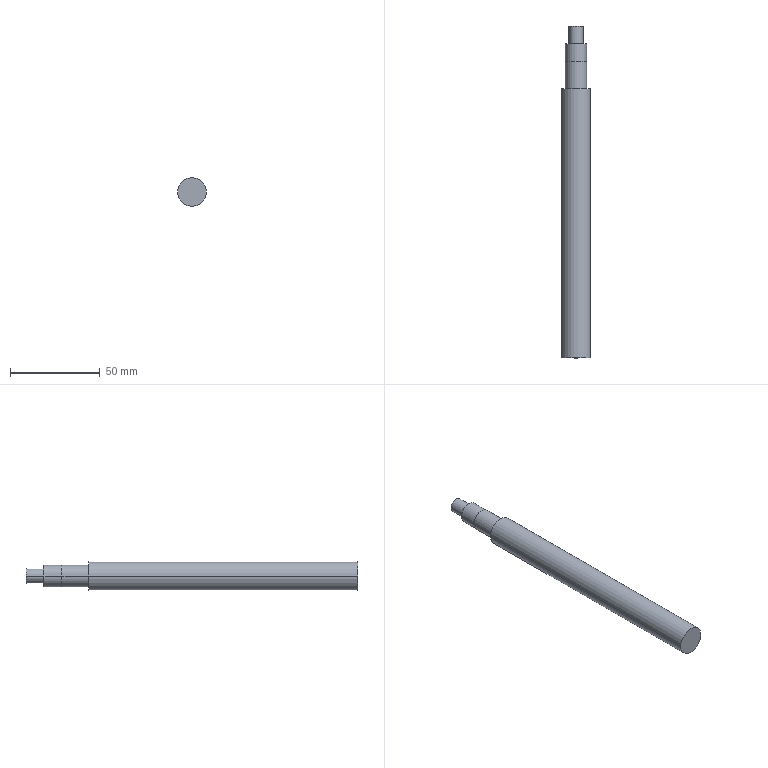Component | SolidWorks | FeedingPressingScrew1-1-1 | 1 solid | 13 faces | box 16 x 185 x 16 mm | volume 33452 mm3 | cylinder 8 | plane 5 | commonest cylinder face diameters 8 x2 11.8 x2 12 x2 16 x2
build123d program:
from build123d import *

# Parameters (mm, degrees)
SKETCH1_R           = 8
BOSS_EXTRUDE1_DEPTH = 150
SKETCH2_R           = 6
BOSS_EXTRUDE2_DEPTH = 15
SKETCH3_R           = 5.9
BOSS_EXTRUDE3_DEPTH = 10
SKETCH4_R           = 4
BOSS_EXTRUDE4_DEPTH = 10


with BuildPart() as part:
    # Sketch1 → Boss-Extrude1 (new body)
    with BuildSketch(Plane.XY):
        Circle(SKETCH1_R)
    extrude(amount=BOSS_EXTRUDE1_DEPTH)

    # Sketch2 → Boss-Extrude2 (add)
    with BuildSketch(Plane.XY.offset(150)):
        with Locations(Location((0, 0, 0), (0, 0, 180))):
            Circle(SKETCH2_R)
    extrude(amount=BOSS_EXTRUDE2_DEPTH)

    # Sketch3 → Boss-Extrude3 (add)
    with BuildSketch(Plane.XY.offset(165)):
        Circle(SKETCH3_R)
    extrude(amount=BOSS_EXTRUDE3_DEPTH)

    # Sketch4 → Boss-Extrude4 (add)
    with BuildSketch(Plane.XY.offset(175)):
        Circle(SKETCH4_R)
    extrude(amount=BOSS_EXTRUDE4_DEPTH)


solid = part.part

# Placed as in the assembly
solid = solid.moved(Location((4.873, 348, 588.209), (-90, 0, 0)))
STEP:
#1=COLOUR_RGB('',0.7922,0.8196,0.9333);
#2=FILL_AREA_STYLE_COLOUR('',#1);
#3=FILL_AREA_STYLE('',(#2));
#4=SURFACE_STYLE_FILL_AREA(#3);
#5=SURFACE_SIDE_STYLE('',(#4));
#6=SURFACE_STYLE_USAGE(.BOTH.,#5);
#7=PRESENTATION_STYLE_ASSIGNMENT((#6));
#8=CARTESIAN_POINT('',(0.3493,20.984,23.158));
#9=VERTEX_POINT('',#8);
#10=CARTESIAN_POINT('',(0.03438,20.984,23.158));
#11=VERTEX_POINT('',#10);
#12=CARTESIAN_POINT('',(0.1919,20.984,23.158));
#13=DIRECTION('',(0.,1.,0.));
#14=DIRECTION('',(1.,0.,0.));
#15=AXIS2_PLACEMENT_3D('',#12,#13,#14);
#16=CIRCLE('',#15,0.1575);
#17=EDGE_CURVE('',#9,#11,#16,.T.);
#18=ORIENTED_EDGE('',*,*,#17,.F.);
#19=CARTESIAN_POINT('',(0.3493,20.591,23.158));
#20=VERTEX_POINT('',#19);
#21=CARTESIAN_POINT('',(0.3493,20.984,23.158));
#22=DIRECTION('',(-0.,-1.,-0.));
#23=VECTOR('',#22,39.37);
#24=LINE('',#21,#23);
#25=EDGE_CURVE('',#9,#20,#24,.T.);
#26=ORIENTED_EDGE('',*,*,#25,.T.);
#27=CARTESIAN_POINT('',(0.03438,20.591,23.158));
#28=VERTEX_POINT('',#27);
#29=CARTESIAN_POINT('',(0.1919,20.591,23.158));
#30=DIRECTION('',(0.,1.,0.));
#31=DIRECTION('',(1.,0.,0.));
#32=AXIS2_PLACEMENT_3D('',#29,#30,#31);
#33=CIRCLE('',#32,0.1575);
#34=EDGE_CURVE('',#20,#28,#33,.T.);
#35=ORIENTED_EDGE('',*,*,#34,.T.);
#36=CARTESIAN_POINT('',(0.03438,20.984,23.158));
#37=DIRECTION('',(-0.,-1.,-0.));
#38=VECTOR('',#37,39.37);
#39=LINE('',#36,#38);
#40=EDGE_CURVE('',#11,#28,#39,.T.);
#41=ORIENTED_EDGE('',*,*,#40,.F.);
#42=EDGE_LOOP('',(#18,#26,#35,#41));
#43=FACE_OUTER_BOUND('',#42,.T.);
#44=CARTESIAN_POINT('',(0.1919,20.984,23.158));
#45=DIRECTION('',(-0.,-1.,-0.));
#46=DIRECTION('',(-1.,0.,0.));
#47=AXIS2_PLACEMENT_3D('',#44,#45,#46);
#48=CYLINDRICAL_SURFACE('',#47,0.1575);
#49=ADVANCED_FACE('',(#43),#48,.T.);
#50=CARTESIAN_POINT('',(0.4241,20.591,23.158));
#51=VERTEX_POINT('',#50);
#52=CARTESIAN_POINT('',(-0.04043,20.591,23.158));
#53=VERTEX_POINT('',#52);
#54=CARTESIAN_POINT('',(0.1919,20.591,23.158));
#55=DIRECTION('',(0.,1.,0.));
#56=DIRECTION('',(1.,0.,0.));
#57=AXIS2_PLACEMENT_3D('',#54,#55,#56);
#58=CIRCLE('',#57,0.2323);
#59=EDGE_CURVE('',#51,#53,#58,.T.);
#60=ORIENTED_EDGE('',*,*,#59,.F.);
#61=CARTESIAN_POINT('',(0.4241,20.197,23.158));
#62=VERTEX_POINT('',#61);
#63=CARTESIAN_POINT('',(0.4241,20.591,23.158));
#64=DIRECTION('',(-0.,-1.,-0.));
#65=VECTOR('',#64,39.37);
#66=LINE('',#63,#65);
#67=EDGE_CURVE('',#51,#62,#66,.T.);
#68=ORIENTED_EDGE('',*,*,#67,.T.);
#69=CARTESIAN_POINT('',(-0.04043,20.197,23.158));
#70=VERTEX_POINT('',#69);
#71=CARTESIAN_POINT('',(0.1919,20.197,23.158));
#72=DIRECTION('',(0.,1.,0.));
#73=DIRECTION('',(1.,0.,0.));
#74=AXIS2_PLACEMENT_3D('',#71,#72,#73);
#75=CIRCLE('',#74,0.2323);
#76=EDGE_CURVE('',#62,#70,#75,.T.);
#77=ORIENTED_EDGE('',*,*,#76,.T.);
#78=CARTESIAN_POINT('',(-0.04043,20.591,23.158));
#79=DIRECTION('',(-0.,-1.,-0.));
#80=VECTOR('',#79,39.37);
#81=LINE('',#78,#80);
#82=EDGE_CURVE('',#53,#70,#81,.T.);
#83=ORIENTED_EDGE('',*,*,#82,.F.);
#84=EDGE_LOOP('',(#60,#68,#77,#83));
#85=FACE_OUTER_BOUND('',#84,.T.);
#86=CARTESIAN_POINT('',(0.1919,20.591,23.158));
#87=DIRECTION('',(-0.,-1.,-0.));
#88=DIRECTION('',(-1.,0.,0.));
#89=AXIS2_PLACEMENT_3D('',#86,#87,#88);
#90=CYLINDRICAL_SURFACE('',#89,0.2323);
#91=ADVANCED_FACE('',(#85),#90,.T.);
#92=CARTESIAN_POINT('',(0.4281,20.197,23.158));
#93=VERTEX_POINT('',#92);
#94=CARTESIAN_POINT('',(-0.04436,20.197,23.158));
#95=VERTEX_POINT('',#94);
#96=CARTESIAN_POINT('',(0.1919,20.197,23.158));
#97=DIRECTION('',(0.,1.,0.));
#98=DIRECTION('',(1.,0.,0.));
#99=AXIS2_PLACEMENT_3D('',#96,#97,#98);
#100=CIRCLE('',#99,0.2362);
#101=EDGE_CURVE('',#93,#95,#100,.T.);
#102=ORIENTED_EDGE('',*,*,#101,.F.);
#103=CARTESIAN_POINT('',(0.4281,19.606,23.158));
#104=VERTEX_POINT('',#103);
#105=CARTESIAN_POINT('',(0.4281,20.197,23.158));
#106=DIRECTION('',(-0.,-1.,-0.));
#107=VECTOR('',#106,39.37);
#108=LINE('',#105,#107);
#109=EDGE_CURVE('',#93,#104,#108,.T.);
#110=ORIENTED_EDGE('',*,*,#109,.T.);
#111=CARTESIAN_POINT('',(-0.04436,19.606,23.158));
#112=VERTEX_POINT('',#111);
#113=CARTESIAN_POINT('',(0.1919,19.606,23.158));
#114=DIRECTION('',(0.,1.,0.));
#115=DIRECTION('',(1.,0.,0.));
#116=AXIS2_PLACEMENT_3D('',#113,#114,#115);
#117=CIRCLE('',#116,0.2362);
#118=EDGE_CURVE('',#104,#112,#117,.T.);
#119=ORIENTED_EDGE('',*,*,#118,.T.);
#120=CARTESIAN_POINT('',(-0.04436,20.197,23.158));
#121=DIRECTION('',(-0.,-1.,-0.));
#122=VECTOR('',#121,39.37);
#123=LINE('',#120,#122);
#124=EDGE_CURVE('',#95,#112,#123,.T.);
#125=ORIENTED_EDGE('',*,*,#124,.F.);
#126=EDGE_LOOP('',(#102,#110,#119,#125));
#127=FACE_OUTER_BOUND('',#126,.T.);
#128=CARTESIAN_POINT('',(0.1919,20.197,23.158));
#129=DIRECTION('',(-0.,-1.,-0.));
#130=DIRECTION('',(-1.,0.,0.));
#131=AXIS2_PLACEMENT_3D('',#128,#129,#130);
#132=CYLINDRICAL_SURFACE('',#131,0.2362);
#133=ADVANCED_FACE('',(#127),#132,.T.);
#134=CARTESIAN_POINT('',(0.5068,19.606,23.158));
#135=VERTEX_POINT('',#134);
#136=CARTESIAN_POINT('',(-0.1231,19.606,23.158));
#137=VERTEX_POINT('',#136);
#138=CARTESIAN_POINT('',(0.1919,19.606,23.158));
#139=DIRECTION('',(0.,1.,0.));
#140=DIRECTION('',(1.,0.,0.));
#141=AXIS2_PLACEMENT_3D('',#138,#139,#140);
#142=CIRCLE('',#141,0.315);
#143=EDGE_CURVE('',#135,#137,#142,.T.);
#144=ORIENTED_EDGE('',*,*,#143,.F.);
#145=CARTESIAN_POINT('',(0.5068,13.701,23.158));
#146=VERTEX_POINT('',#145);
#147=CARTESIAN_POINT('',(0.5068,19.606,23.158));
#148=DIRECTION('',(-0.,-1.,-0.));
#149=VECTOR('',#148,39.37);
#150=LINE('',#147,#149);
#151=EDGE_CURVE('',#135,#146,#150,.T.);
#152=ORIENTED_EDGE('',*,*,#151,.T.);
#153=CARTESIAN_POINT('',(-0.1231,13.701,23.158));
#154=VERTEX_POINT('',#153);
#155=CARTESIAN_POINT('',(0.1919,13.701,23.158));
#156=DIRECTION('',(0.,1.,0.));
#157=DIRECTION('',(1.,0.,0.));
#158=AXIS2_PLACEMENT_3D('',#155,#156,#157);
#159=CIRCLE('',#158,0.315);
#160=EDGE_CURVE('',#146,#154,#159,.T.);
#161=ORIENTED_EDGE('',*,*,#160,.T.);
#162=CARTESIAN_POINT('',(-0.1231,19.606,23.158));
#163=DIRECTION('',(-0.,-1.,-0.));
#164=VECTOR('',#163,39.37);
#165=LINE('',#162,#164);
#166=EDGE_CURVE('',#137,#154,#165,.T.);
#167=ORIENTED_EDGE('',*,*,#166,.F.);
#168=EDGE_LOOP('',(#144,#152,#161,#167));
#169=FACE_OUTER_BOUND('',#168,.T.);
#170=CARTESIAN_POINT('',(0.1919,19.606,23.158));
#171=DIRECTION('',(-0.,-1.,-0.));
#172=DIRECTION('',(-1.,0.,0.));
#173=AXIS2_PLACEMENT_3D('',#170,#171,#172);
#174=CYLINDRICAL_SURFACE('',#173,0.315);
#175=ADVANCED_FACE('',(#169),#174,.T.);
#176=ORIENTED_EDGE('',*,*,#151,.F.);
#177=CARTESIAN_POINT('',(0.1919,19.606,23.158));
#178=DIRECTION('',(0.,1.,0.));
#179=DIRECTION('',(1.,0.,0.));
#180=AXIS2_PLACEMENT_3D('',#177,#178,#179);
#181=CIRCLE('',#180,0.315);
#182=EDGE_CURVE('',#137,#135,#181,.T.);
#183=ORIENTED_EDGE('',*,*,#182,.F.);
#184=ORIENTED_EDGE('',*,*,#166,.T.);
#185=CARTESIAN_POINT('',(0.1919,13.701,23.158));
#186=DIRECTION('',(0.,1.,0.));
#187=DIRECTION('',(1.,0.,0.));
#188=AXIS2_PLACEMENT_3D('',#185,#186,#187);
#189=CIRCLE('',#188,0.315);
#190=EDGE_CURVE('',#154,#146,#189,.T.);
#191=ORIENTED_EDGE('',*,*,#190,.T.);
#192=EDGE_LOOP('',(#176,#183,#184,#191));
#193=FACE_OUTER_BOUND('',#192,.T.);
#194=CARTESIAN_POINT('',(0.1919,19.606,23.158));
#195=DIRECTION('',(-0.,-1.,-0.));
#196=DIRECTION('',(-1.,0.,0.));
#197=AXIS2_PLACEMENT_3D('',#194,#195,#196);
#198=CYLINDRICAL_SURFACE('',#197,0.315);
#199=ADVANCED_FACE('',(#193),#198,.T.);
#200=CARTESIAN_POINT('',(0.1919,19.606,23.158));
#201=DIRECTION('',(0.,1.,0.));
#202=DIRECTION('',(1.,0.,0.));
#203=AXIS2_PLACEMENT_3D('',#200,#201,#202);
#204=CIRCLE('',#203,0.2362);
#205=EDGE_CURVE('',#112,#104,#204,.T.);
#206=ORIENTED_EDGE('',*,*,#205,.F.);
#207=ORIENTED_EDGE('',*,*,#118,.F.);
#208=EDGE_LOOP('',(#206,#207));
#209=FACE_BOUND('',#208,.T.);
#210=ORIENTED_EDGE('',*,*,#182,.T.);
#211=ORIENTED_EDGE('',*,*,#143,.T.);
#212=EDGE_LOOP('',(#210,#211));
#213=FACE_OUTER_BOUND('',#212,.T.);
#214=CARTESIAN_POINT('',(0.1919,19.606,23.158));
#215=DIRECTION('',(0.,1.,0.));
#216=DIRECTION('',(1.,-0.,-0.));
#217=AXIS2_PLACEMENT_3D('',#214,#215,#216);
#218=PLANE('',#217);
#219=ADVANCED_FACE('',(#209,#213),#218,.T.);
#220=ORIENTED_EDGE('',*,*,#190,.F.);
#221=ORIENTED_EDGE('',*,*,#160,.F.);
#222=EDGE_LOOP('',(#220,#221));
#223=FACE_OUTER_BOUND('',#222,.T.);
#224=CARTESIAN_POINT('',(0.1919,13.701,23.158));
#225=DIRECTION('',(0.,1.,0.));
#226=DIRECTION('',(1.,-0.,-0.));
#227=AXIS2_PLACEMENT_3D('',#224,#225,#226);
#228=PLANE('',#227);
#229=ADVANCED_FACE('',(#223),#228,.F.);
#230=ORIENTED_EDGE('',*,*,#109,.F.);
#231=CARTESIAN_POINT('',(0.1919,20.197,23.158));
#232=DIRECTION('',(0.,1.,0.));
#233=DIRECTION('',(1.,0.,0.));
#234=AXIS2_PLACEMENT_3D('',#231,#232,#233);
#235=CIRCLE('',#234,0.2362);
#236=EDGE_CURVE('',#95,#93,#235,.T.);
#237=ORIENTED_EDGE('',*,*,#236,.F.);
#238=ORIENTED_EDGE('',*,*,#124,.T.);
#239=ORIENTED_EDGE('',*,*,#205,.T.);
#240=EDGE_LOOP('',(#230,#237,#238,#239));
#241=FACE_OUTER_BOUND('',#240,.T.);
#242=CARTESIAN_POINT('',(0.1919,20.197,23.158));
#243=DIRECTION('',(-0.,-1.,-0.));
#244=DIRECTION('',(-1.,0.,0.));
#245=AXIS2_PLACEMENT_3D('',#242,#243,#244);
#246=CYLINDRICAL_SURFACE('',#245,0.2362);
#247=ADVANCED_FACE('',(#241),#246,.T.);
#248=CARTESIAN_POINT('',(0.1919,20.197,23.158));
#249=DIRECTION('',(0.,1.,0.));
#250=DIRECTION('',(1.,0.,0.));
#251=AXIS2_PLACEMENT_3D('',#248,#249,#250);
#252=CIRCLE('',#251,0.2323);
#253=EDGE_CURVE('',#70,#62,#252,.T.);
#254=ORIENTED_EDGE('',*,*,#253,.F.);
#255=ORIENTED_EDGE('',*,*,#76,.F.);
#256=EDGE_LOOP('',(#254,#255));
#257=FACE_BOUND('',#256,.T.);
#258=ORIENTED_EDGE('',*,*,#236,.T.);
#259=ORIENTED_EDGE('',*,*,#101,.T.);
#260=EDGE_LOOP('',(#258,#259));
#261=FACE_OUTER_BOUND('',#260,.T.);
#262=CARTESIAN_POINT('',(0.1919,20.197,23.158));
#263=DIRECTION('',(0.,1.,0.));
#264=DIRECTION('',(1.,-0.,-0.));
#265=AXIS2_PLACEMENT_3D('',#262,#263,#264);
#266=PLANE('',#265);
#267=ADVANCED_FACE('',(#257,#261),#266,.T.);
#268=ORIENTED_EDGE('',*,*,#67,.F.);
#269=CARTESIAN_POINT('',(0.1919,20.591,23.158));
#270=DIRECTION('',(0.,1.,0.));
#271=DIRECTION('',(1.,0.,0.));
#272=AXIS2_PLACEMENT_3D('',#269,#270,#271);
#273=CIRCLE('',#272,0.2323);
#274=EDGE_CURVE('',#53,#51,#273,.T.);
#275=ORIENTED_EDGE('',*,*,#274,.F.);
#276=ORIENTED_EDGE('',*,*,#82,.T.);
#277=ORIENTED_EDGE('',*,*,#253,.T.);
#278=EDGE_LOOP('',(#268,#275,#276,#277));
#279=FACE_OUTER_BOUND('',#278,.T.);
#280=CARTESIAN_POINT('',(0.1919,20.591,23.158));
#281=DIRECTION('',(-0.,-1.,-0.));
#282=DIRECTION('',(-1.,0.,0.));
#283=AXIS2_PLACEMENT_3D('',#280,#281,#282);
#284=CYLINDRICAL_SURFACE('',#283,0.2323);
#285=ADVANCED_FACE('',(#279),#284,.T.);
#286=CARTESIAN_POINT('',(0.1919,20.591,23.158));
#287=DIRECTION('',(0.,1.,0.));
#288=DIRECTION('',(1.,0.,0.));
#289=AXIS2_PLACEMENT_3D('',#286,#287,#288);
#290=CIRCLE('',#289,0.1575);
#291=EDGE_CURVE('',#28,#20,#290,.T.);
#292=ORIENTED_EDGE('',*,*,#291,.F.);
#293=ORIENTED_EDGE('',*,*,#34,.F.);
#294=EDGE_LOOP('',(#292,#293));
#295=FACE_BOUND('',#294,.T.);
#296=ORIENTED_EDGE('',*,*,#274,.T.);
#297=ORIENTED_EDGE('',*,*,#59,.T.);
#298=EDGE_LOOP('',(#296,#297));
#299=FACE_OUTER_BOUND('',#298,.T.);
#300=CARTESIAN_POINT('',(0.1919,20.591,23.158));
#301=DIRECTION('',(0.,1.,0.));
#302=DIRECTION('',(1.,-0.,-0.));
#303=AXIS2_PLACEMENT_3D('',#300,#301,#302);
#304=PLANE('',#303);
#305=ADVANCED_FACE('',(#295,#299),#304,.T.);
#306=ORIENTED_EDGE('',*,*,#25,.F.);
#307=CARTESIAN_POINT('',(0.1919,20.984,23.158));
#308=DIRECTION('',(0.,1.,0.));
#309=DIRECTION('',(1.,0.,0.));
#310=AXIS2_PLACEMENT_3D('',#307,#308,#309);
#311=CIRCLE('',#310,0.1575);
#312=EDGE_CURVE('',#11,#9,#311,.T.);
#313=ORIENTED_EDGE('',*,*,#312,.F.);
#314=ORIENTED_EDGE('',*,*,#40,.T.);
#315=ORIENTED_EDGE('',*,*,#291,.T.);
#316=EDGE_LOOP('',(#306,#313,#314,#315));
#317=FACE_OUTER_BOUND('',#316,.T.);
#318=CARTESIAN_POINT('',(0.1919,20.984,23.158));
#319=DIRECTION('',(-0.,-1.,-0.));
#320=DIRECTION('',(-1.,0.,0.));
#321=AXIS2_PLACEMENT_3D('',#318,#319,#320);
#322=CYLINDRICAL_SURFACE('',#321,0.1575);
#323=ADVANCED_FACE('',(#317),#322,.T.);
#324=ORIENTED_EDGE('',*,*,#312,.T.);
#325=ORIENTED_EDGE('',*,*,#17,.T.);
#326=EDGE_LOOP('',(#324,#325));
#327=FACE_OUTER_BOUND('',#326,.T.);
#328=CARTESIAN_POINT('',(0.1919,20.984,23.158));
#329=DIRECTION('',(0.,1.,0.));
#330=DIRECTION('',(1.,-0.,-0.));
#331=AXIS2_PLACEMENT_3D('',#328,#329,#330);
#332=PLANE('',#331);
#333=ADVANCED_FACE('',(#327),#332,.T.);
#334=CLOSED_SHELL('',(#49,#91,#133,#175,#199,#219,#229,#247,#267,#285,#305,#323,#333));
#335=MANIFOLD_SOLID_BREP('',#334);
#336=STYLED_ITEM('',(#7),#335);
#337=(LENGTH_UNIT()NAMED_UNIT(*)SI_UNIT($,.METRE.));
#338=LENGTH_MEASURE_WITH_UNIT(LENGTH_MEASURE(0.0254),#337);
#339=DIMENSIONAL_EXPONENTS(1.,0.,0.,0.,0.,0.,0.);
#340=(CONVERSION_BASED_UNIT('',#338)LENGTH_UNIT()NAMED_UNIT(#339));
#341=UNCERTAINTY_MEASURE_WITH_UNIT(LENGTH_MEASURE(0.00001),#340,'','');
#342=(NAMED_UNIT(*)PLANE_ANGLE_UNIT()SI_UNIT($,.RADIAN.));
#343=(NAMED_UNIT(*)SI_UNIT($,.STERADIAN.)SOLID_ANGLE_UNIT());
#344=(GEOMETRIC_REPRESENTATION_CONTEXT(3)GLOBAL_UNCERTAINTY_ASSIGNED_CONTEXT((#341))GLOBAL_UNIT_ASSIGNED_CONTEXT((#340,#342,#343))REPRESENTATION_CONTEXT('',''));
#345=MECHANICAL_DESIGN_GEOMETRIC_PRESENTATION_REPRESENTATION('',(#336),#344);
#346=CARTESIAN_POINT('',(0.,0.,0.));
#347=DIRECTION('',(0.,0.,1.));
#348=DIRECTION('',(1.,0.,0.));
#349=AXIS2_PLACEMENT_3D('',#346,#347,#348);
#350=(LENGTH_UNIT()NAMED_UNIT(*)SI_UNIT($,.METRE.));
#351=LENGTH_MEASURE_WITH_UNIT(LENGTH_MEASURE(0.0254),#350);
#352=DIMENSIONAL_EXPONENTS(1.,0.,0.,0.,0.,0.,0.);
#353=(CONVERSION_BASED_UNIT('',#351)LENGTH_UNIT()NAMED_UNIT(#352));
#354=UNCERTAINTY_MEASURE_WITH_UNIT(LENGTH_MEASURE(0.00001),#353,'','');
#355=(NAMED_UNIT(*)PLANE_ANGLE_UNIT()SI_UNIT($,.RADIAN.));
#356=(NAMED_UNIT(*)SI_UNIT($,.STERADIAN.)SOLID_ANGLE_UNIT());
#357=(GEOMETRIC_REPRESENTATION_CONTEXT(3)GLOBAL_UNCERTAINTY_ASSIGNED_CONTEXT((#354))GLOBAL_UNIT_ASSIGNED_CONTEXT((#353,#355,#356))REPRESENTATION_CONTEXT('',''));
#358=ADVANCED_BREP_SHAPE_REPRESENTATION('',(#335,#349),#357);
#359=PRESENTATION_LAYER_ASSIGNMENT('','',(#336));